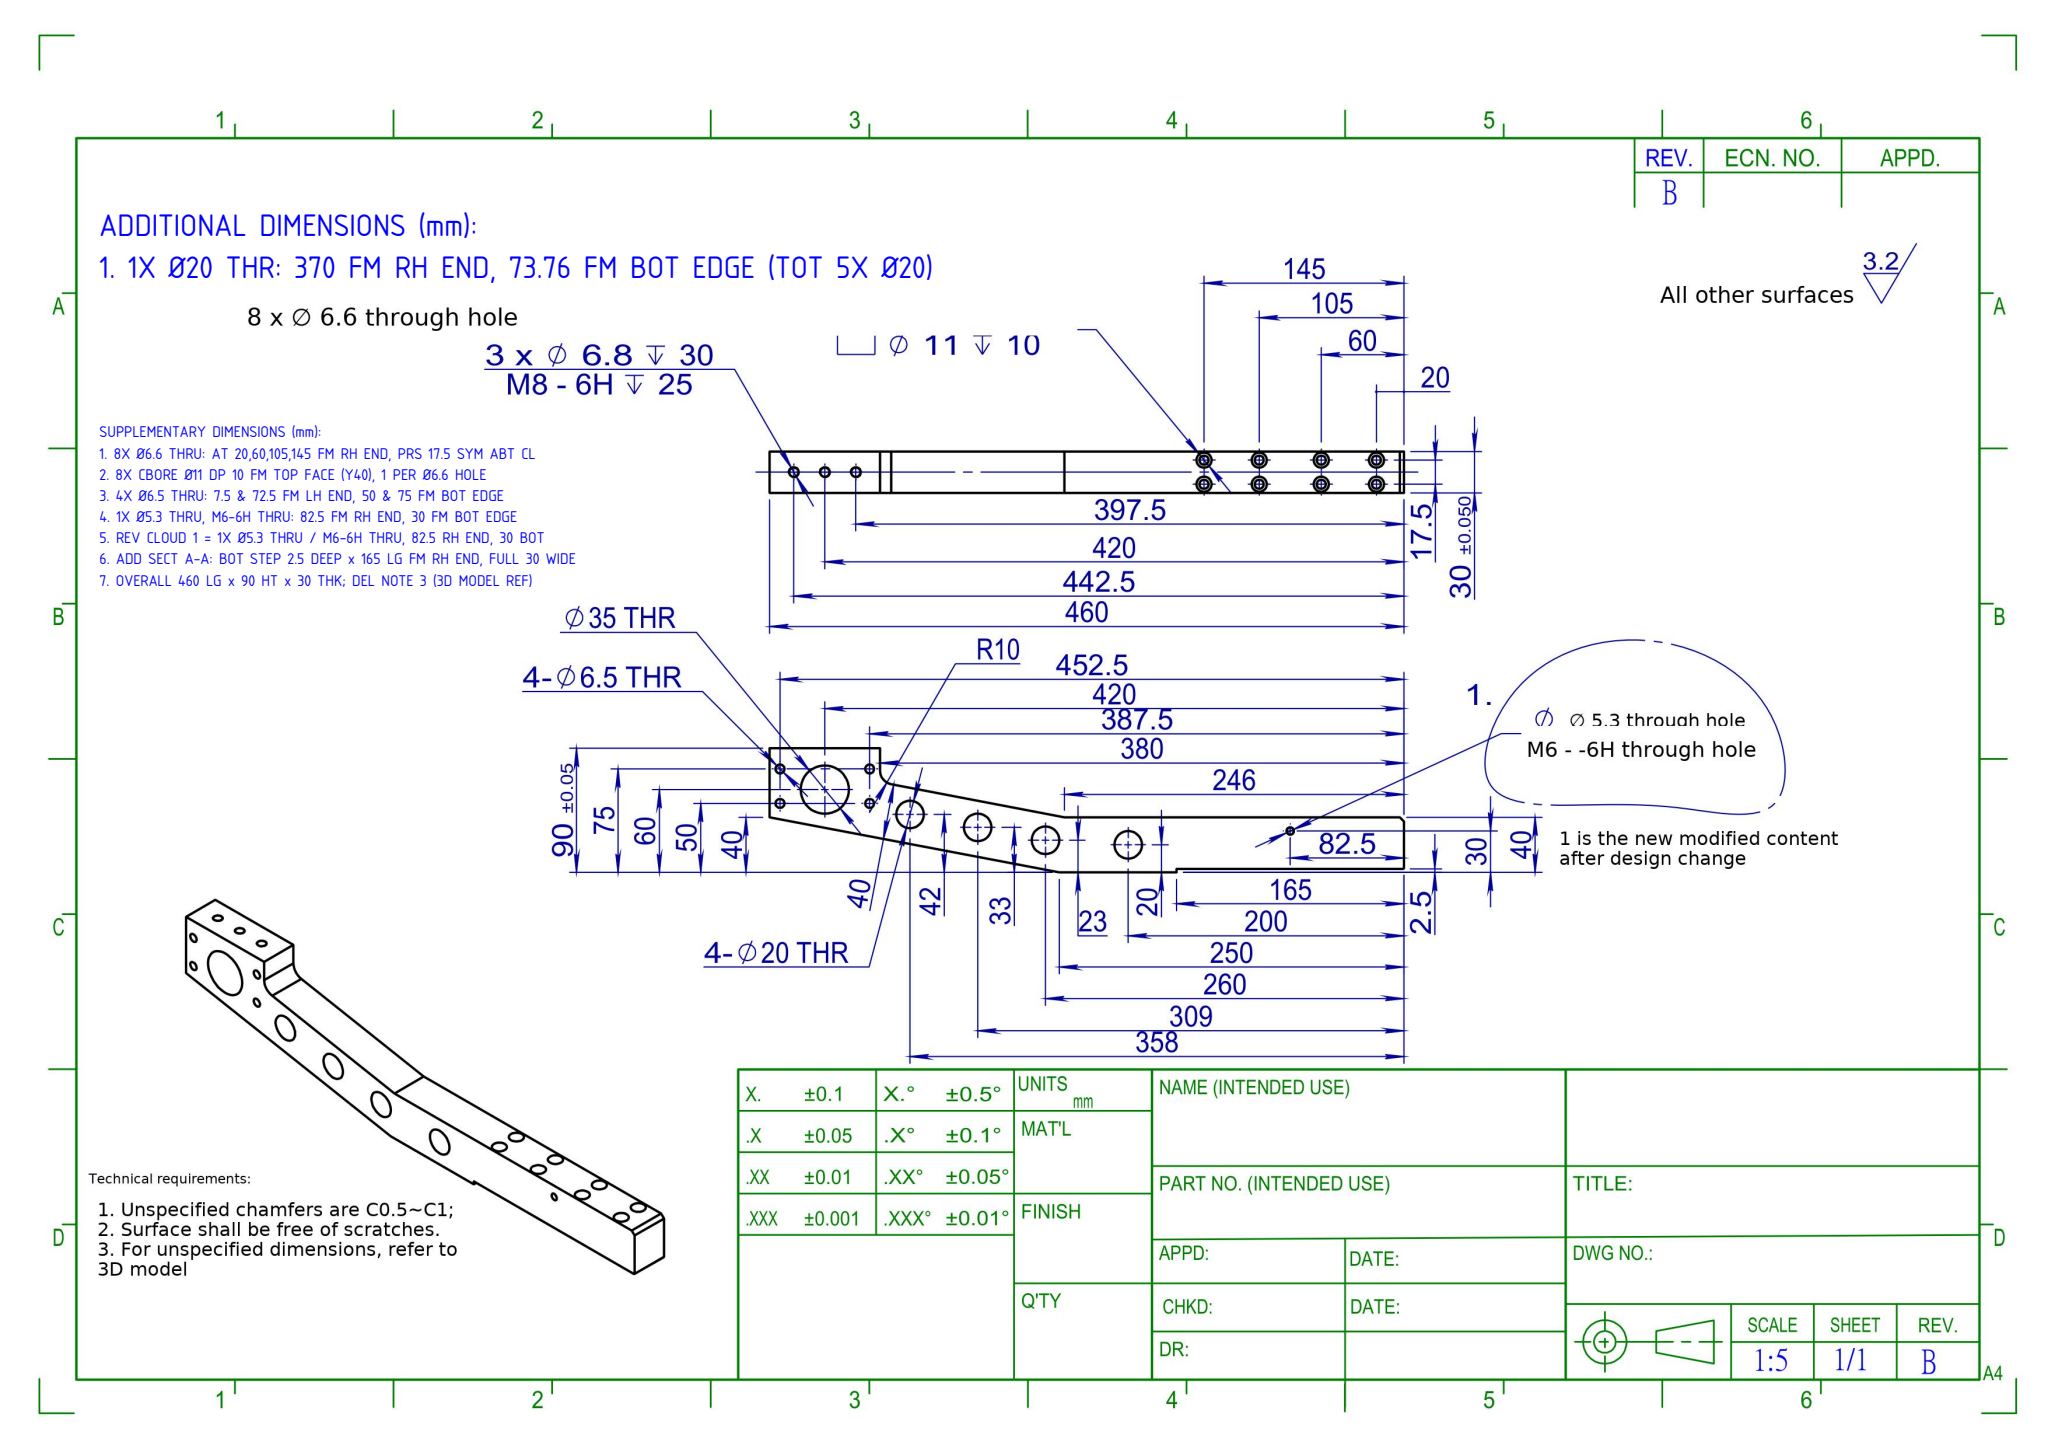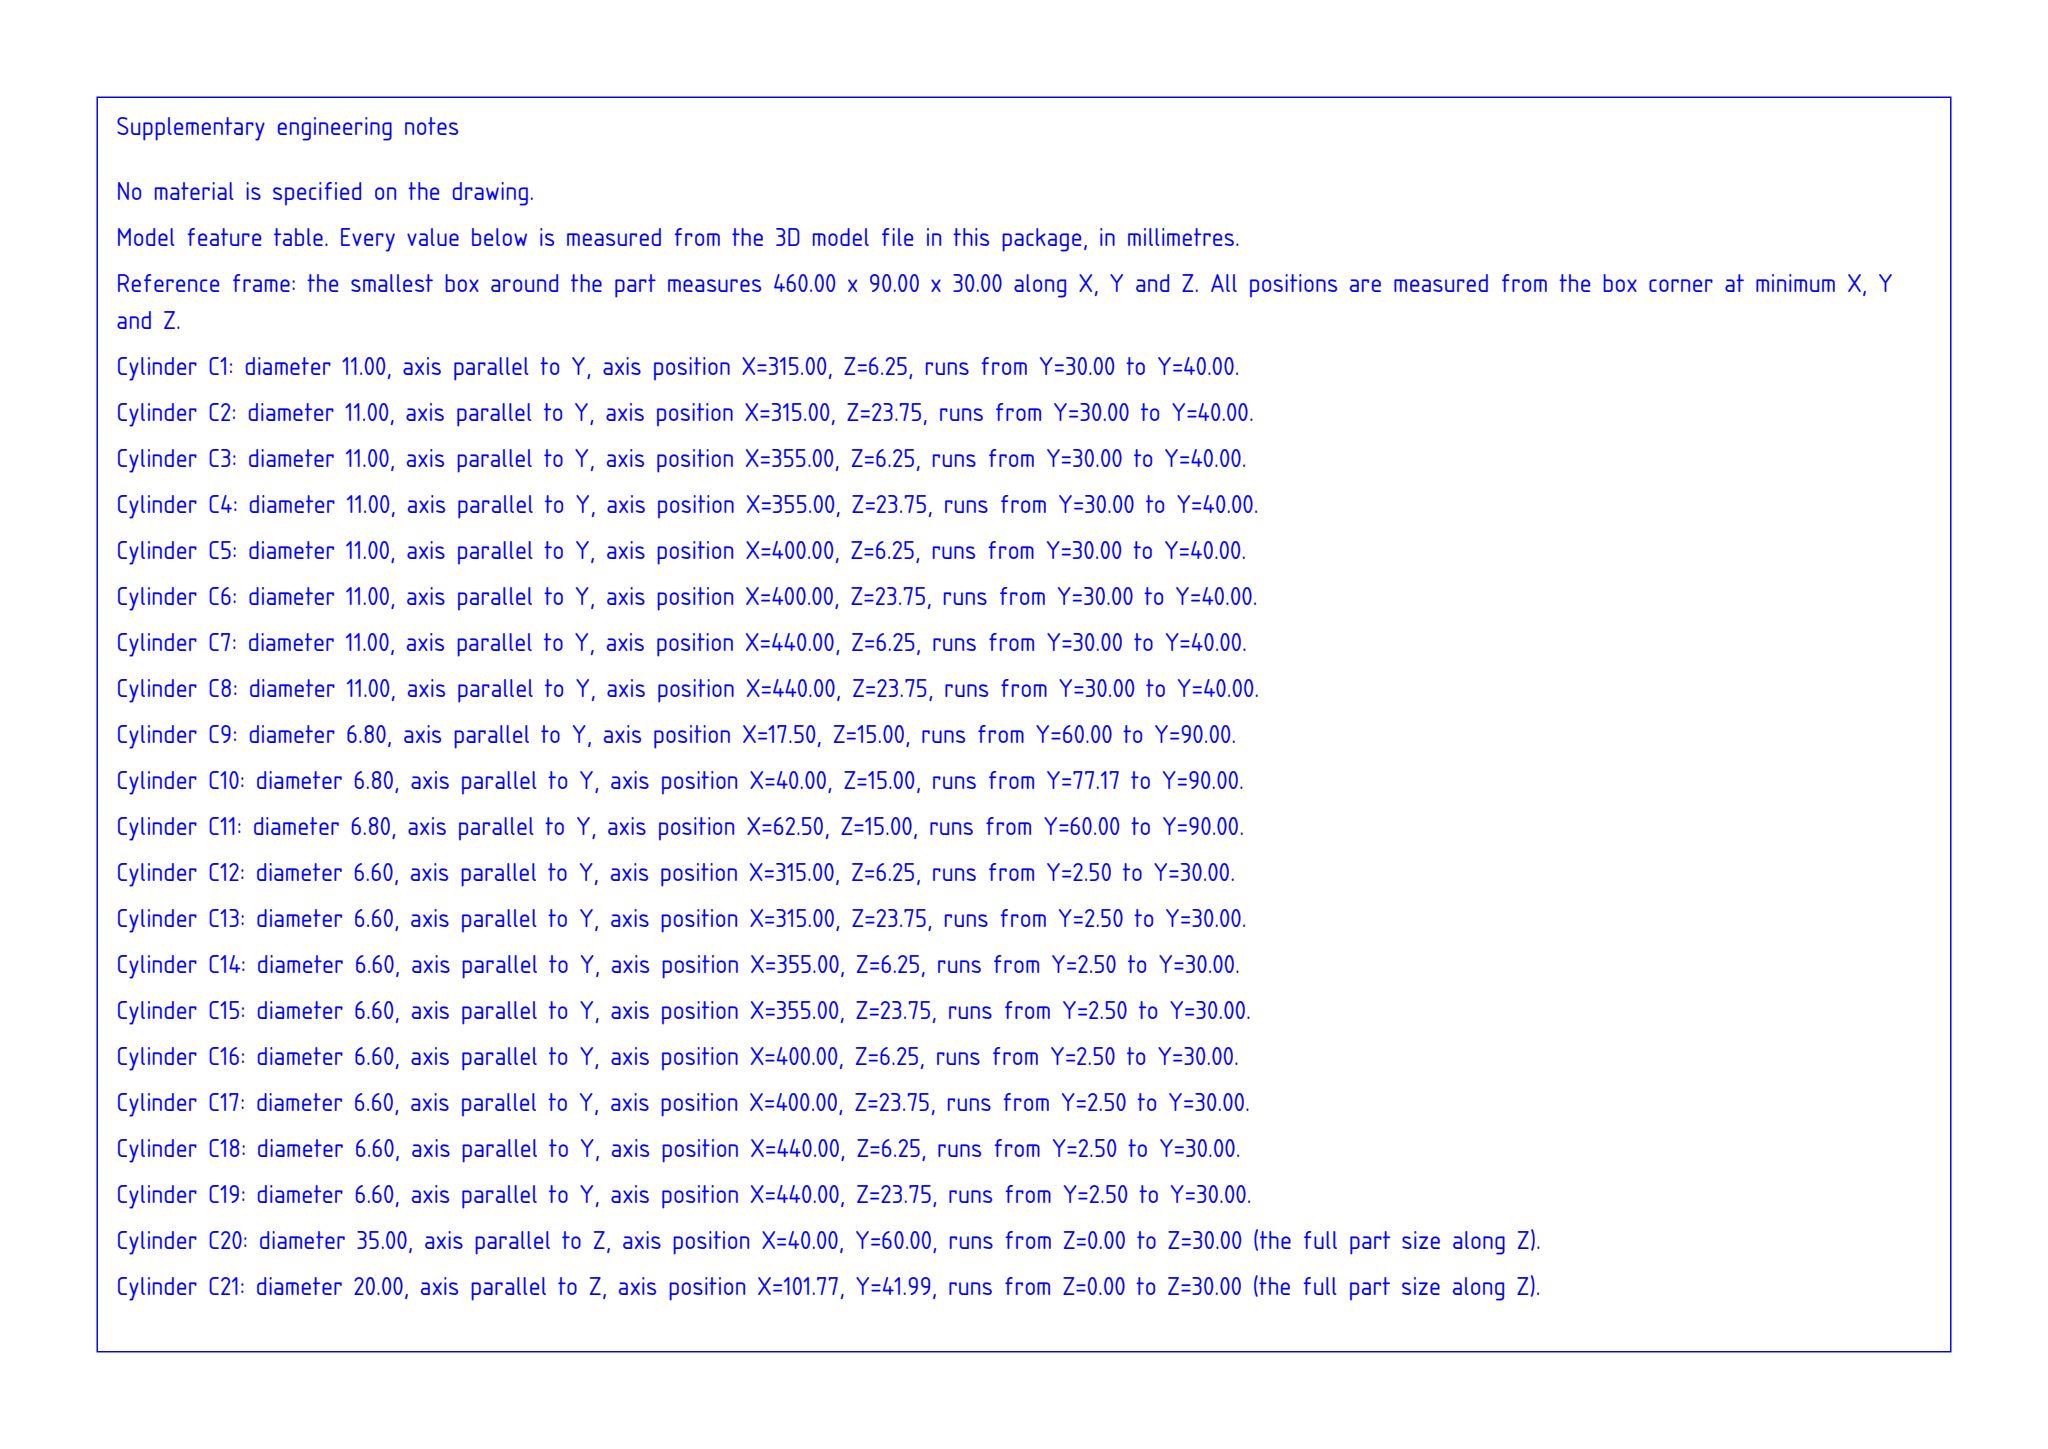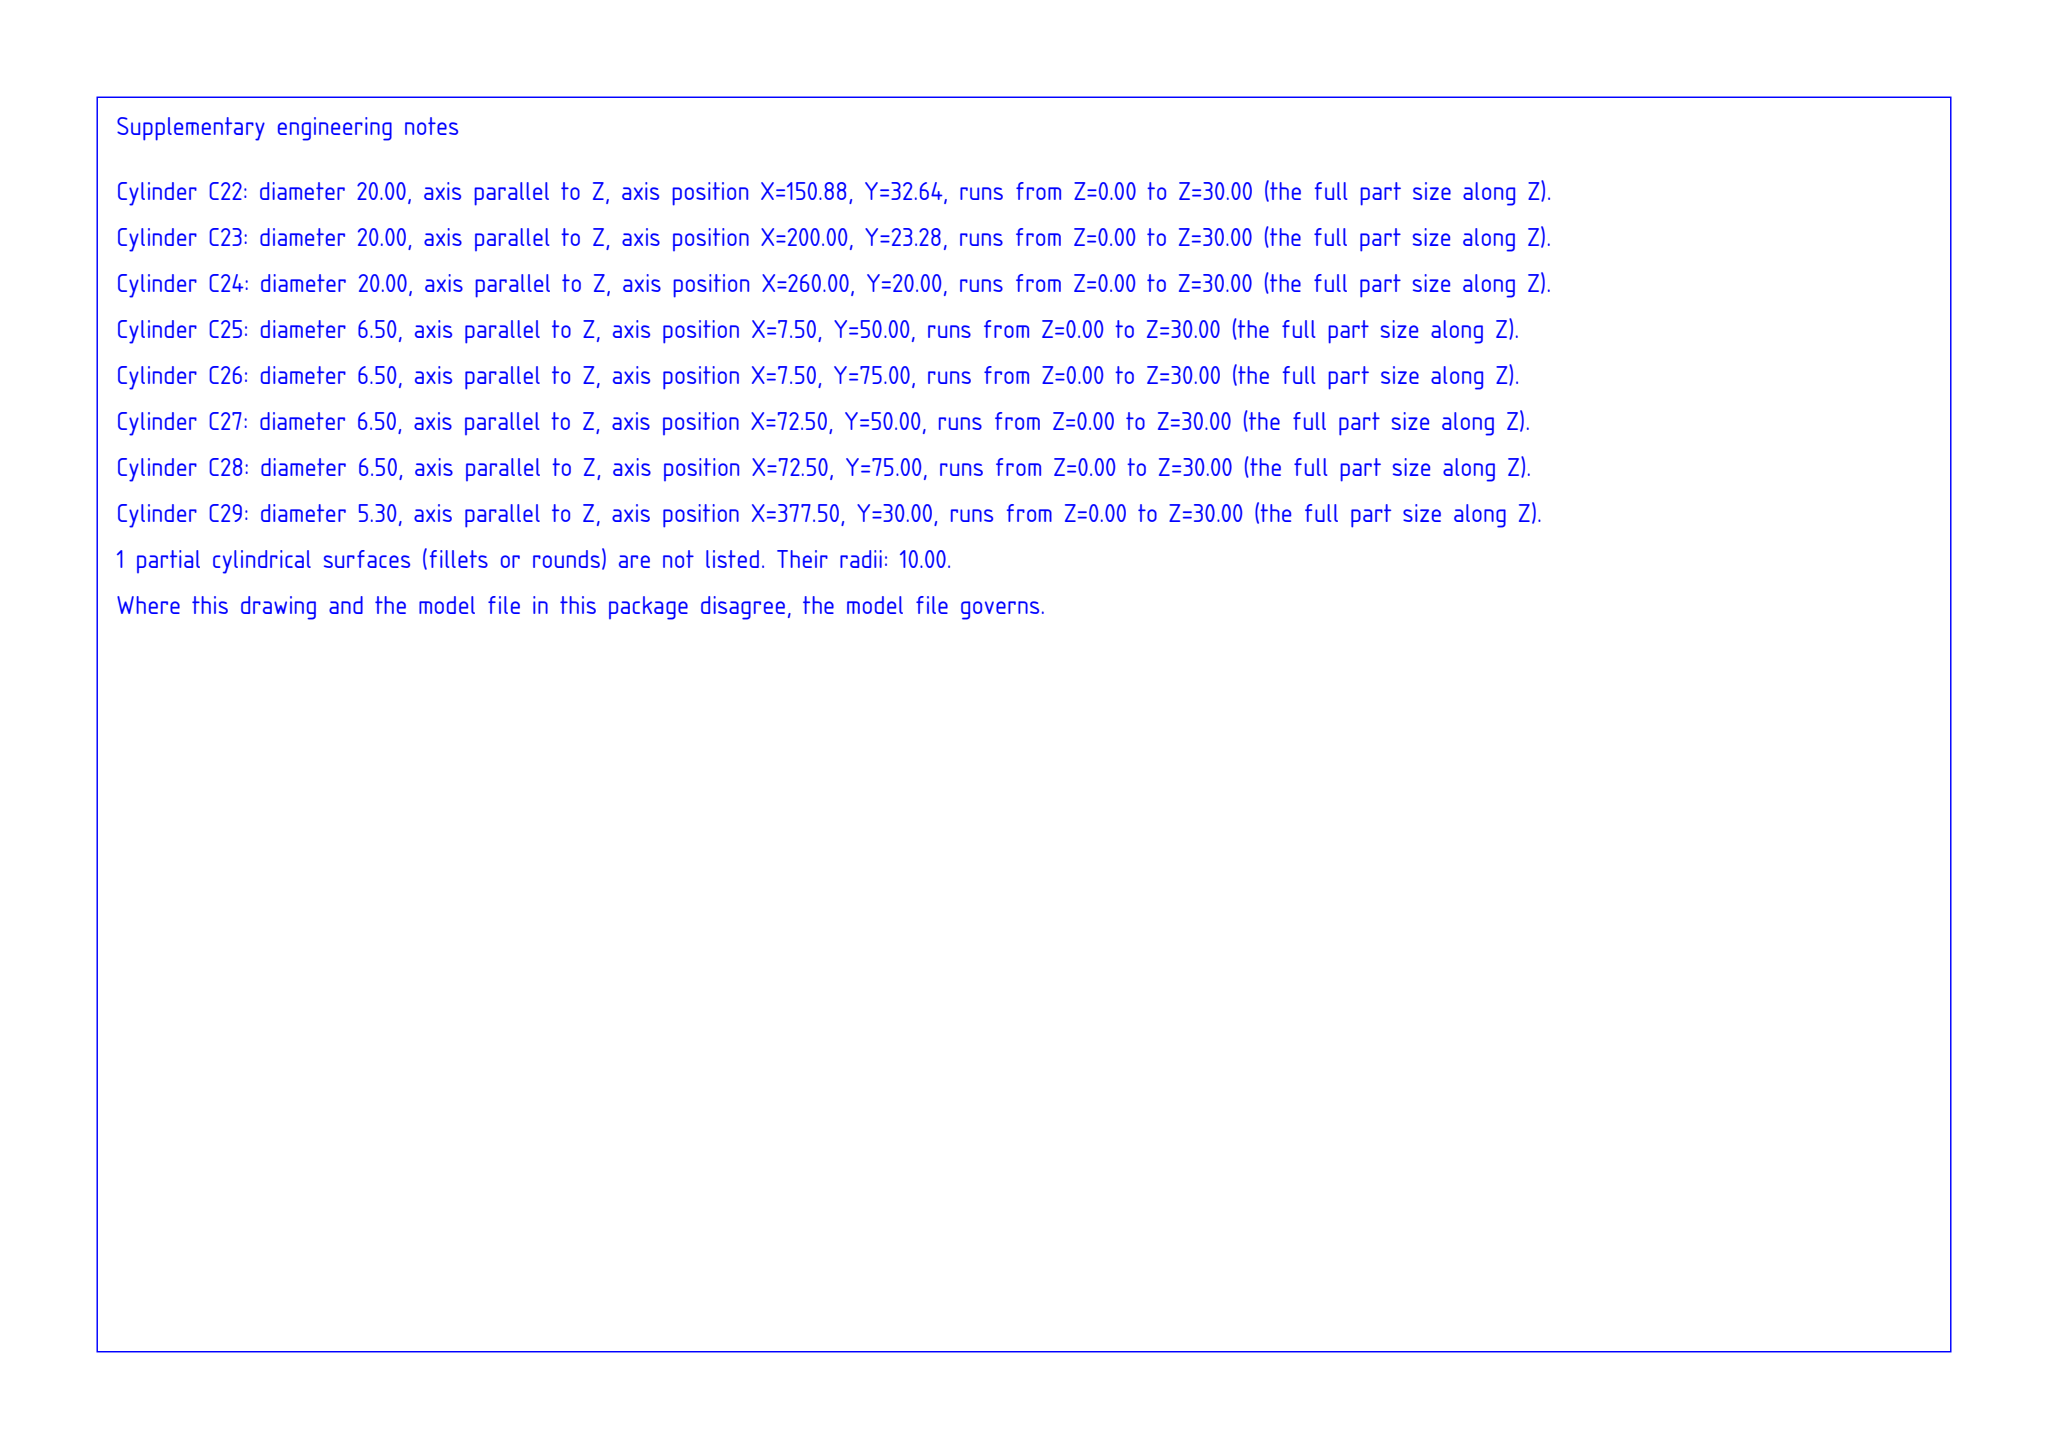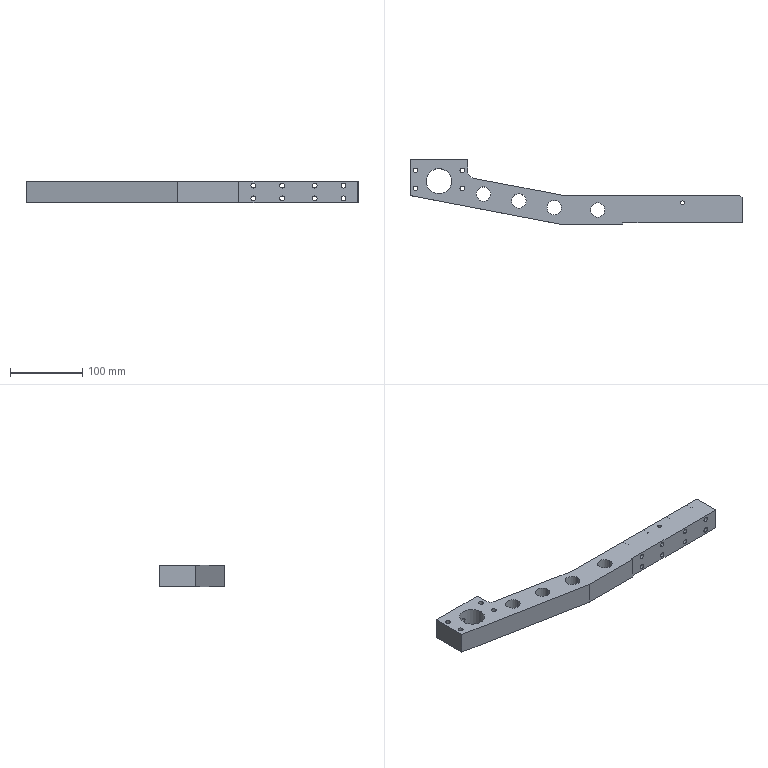Part | SolidWorks | mm | 1 solid | 85 faces | box 460 x 90 x 30 mm | volume 496005 mm3 | cylinder 59 | plane 22 | cone 4 | commonest cylinder face diameters 11 x16 6.6 x16 20 x9 6.5 x8 6.8 x6 5.3 x2 35 x2
build123d program:
from build123d import *

# Parameters (mm, degrees)
BOSS_EXTRUDE1_DEPTH                                  = 15
SKETCH2_R                                            = 10
CUT_EXTRUDE1_DEPTH                                   = 470.681
CHAMFER1_SIZE                                        = 3
SKETCH3_R                                            = 3.25
CUT_EXTRUDE2_DEPTH                                   = 470.681
M8_TAPPED_HOLE1_D                                    = 6.8
M8_TAPPED_HOLE1_DEPTH                                = 30
M8_TAPPED_HOLE1_TIP                                  = 2.043
SKETCH6_W                                            = 165
SKETCH6_H                                            = 2.5
CUT_EXTRUDE3_DEPTH                                   = 470.681
COUNTERBORE_FOR_M6_HEX_SOCKET_HEAD_CAP_S_D           = 6.6
COUNTERBORE_FOR_M6_HEX_SOCKET_HEAD_CAP_S_CBORE_D     = 11
COUNTERBORE_FOR_M6_HEX_SOCKET_HEAD_CAP_S_CBORE_DEPTH = 10
SKETCH10_R                                           = 17.5
CUT_EXTRUDE5_DEPTH                                   = 470.681
FILLET1_R                                            = 10
M6_TAPPED_HOLE1_D                                    = 5.3


with BuildPart() as part:
    # Sketch1 → Boss-Extrude1 (new, symmetric)
    with BuildSketch(Plane.XY):
        Polygon((0, 0), (0, -50), (210, -90), (460, -90), (460, -50), (213.776, -50), (80, -24.519), (80, 0), align=None)
    extrude(amount=BOSS_EXTRUDE1_DEPTH, both=True)

    # Sketch2 → Cut-Extrude1 (cut, through all)
    with BuildSketch(Plane.XY.offset(15)):
        with Locations((101.766, -48.006)):
            Circle(SKETCH2_R)
        with Locations((150.883, -57.362)):
            Circle(SKETCH2_R)
        with Locations((200, -66.718)):
            Circle(SKETCH2_R)
        with Locations((260, -70)):
            Circle(SKETCH2_R)
    extrude(amount=-CUT_EXTRUDE1_DEPTH, mode=Mode.SUBTRACT)

    # Chamfer1
    chamfer1_edges = [part.edges().sort_by_distance(p)[0] for p in [
        (460, -50, 0),
        (460, -90, 0),
    ]]
    chamfer(chamfer1_edges, length=CHAMFER1_SIZE)

    # Sketch3 → Cut-Extrude2 (cut, through all)
    with BuildSketch(Plane(origin=(0, 0, -15), x_dir=(-1, 0, 0), z_dir=(0, 0, -1))):
        with Locations((-72.5, -15)):
            Circle(SKETCH3_R)
        with Locations((-72.5, -40)):
            Circle(SKETCH3_R)
        with Locations((-7.5, -15)):
            Circle(SKETCH3_R)
        with Locations((-7.5, -40)):
            Circle(SKETCH3_R)
    extrude(amount=-CUT_EXTRUDE2_DEPTH, mode=Mode.SUBTRACT)

    # M8 Tapped Hole1
    with Locations(Plane(origin=(0, 0, 0), x_dir=(1, 0, 0), z_dir=(0, 1, 0))):
        with Locations((17.5, 0), (40, 0), (62.5, 0)):
            Hole(M8_TAPPED_HOLE1_D / 2, depth=M8_TAPPED_HOLE1_DEPTH)
            with Locations((0, 0, -(M8_TAPPED_HOLE1_DEPTH + M8_TAPPED_HOLE1_TIP / 2))):  # 118° drill point
                Cone(0, M8_TAPPED_HOLE1_D / 2, M8_TAPPED_HOLE1_TIP, mode=Mode.SUBTRACT)

    # Sketch6 → Cut-Extrude3 (cut, through all)
    with BuildSketch(Plane.XY.offset(15)):
        with Locations((377.5, -88.75)):
            Rectangle(SKETCH6_W, SKETCH6_H)
    extrude(amount=-CUT_EXTRUDE3_DEPTH, mode=Mode.SUBTRACT)

    # Counterbore for M6 Hex Socket Head Cap S (through all)
    with Locations(Plane(origin=(0, -50, 0), x_dir=(1, 0, 0), z_dir=(0, 1, 0))):
        with Locations((355, 8.75), (355, -8.75), (315, 8.75), (315, -8.75), (400, 8.75), (400, -8.75), (440, 8.75), (440, -8.75)):
            CounterBoreHole(COUNTERBORE_FOR_M6_HEX_SOCKET_HEAD_CAP_S_D / 2, COUNTERBORE_FOR_M6_HEX_SOCKET_HEAD_CAP_S_CBORE_D / 2, COUNTERBORE_FOR_M6_HEX_SOCKET_HEAD_CAP_S_CBORE_DEPTH)

    # Sketch10 → Cut-Extrude5 (cut, through all)
    with BuildSketch(Plane(origin=(0, 0, -15), x_dir=(-1, 0, 0), z_dir=(0, 0, -1))):
        with Locations((-40, -30)):
            Circle(SKETCH10_R)
    extrude(amount=-CUT_EXTRUDE5_DEPTH, mode=Mode.SUBTRACT)

    # Fillet1
    fillet1_edges = [part.edges().sort_by_distance(p)[0] for p in [
        (80, -24.519, 0),
    ]]
    fillet(fillet1_edges, radius=FILLET1_R)

    # M6 Tapped Hole1 (through all)
    with Locations(Plane.XY.offset(15)):
        with Locations((377.5, -60)):
            Hole(M6_TAPPED_HOLE1_D / 2)


solid = part.part